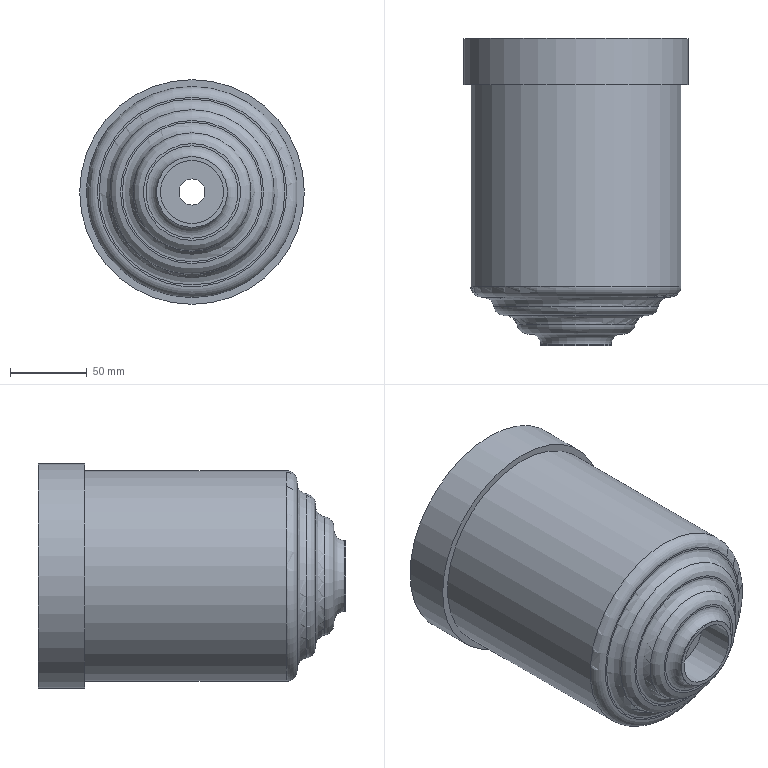Component | NX | HOUSING | 1 solid | 34 faces | volume 1096359 mm3 | cylinder 13 | plane 9 | cone 6 | torus 6 | commonest cylinder face diameters 6 x6 17 x1 41 x1 114 x1 146 x1 137 x1 46 x1 40 x1